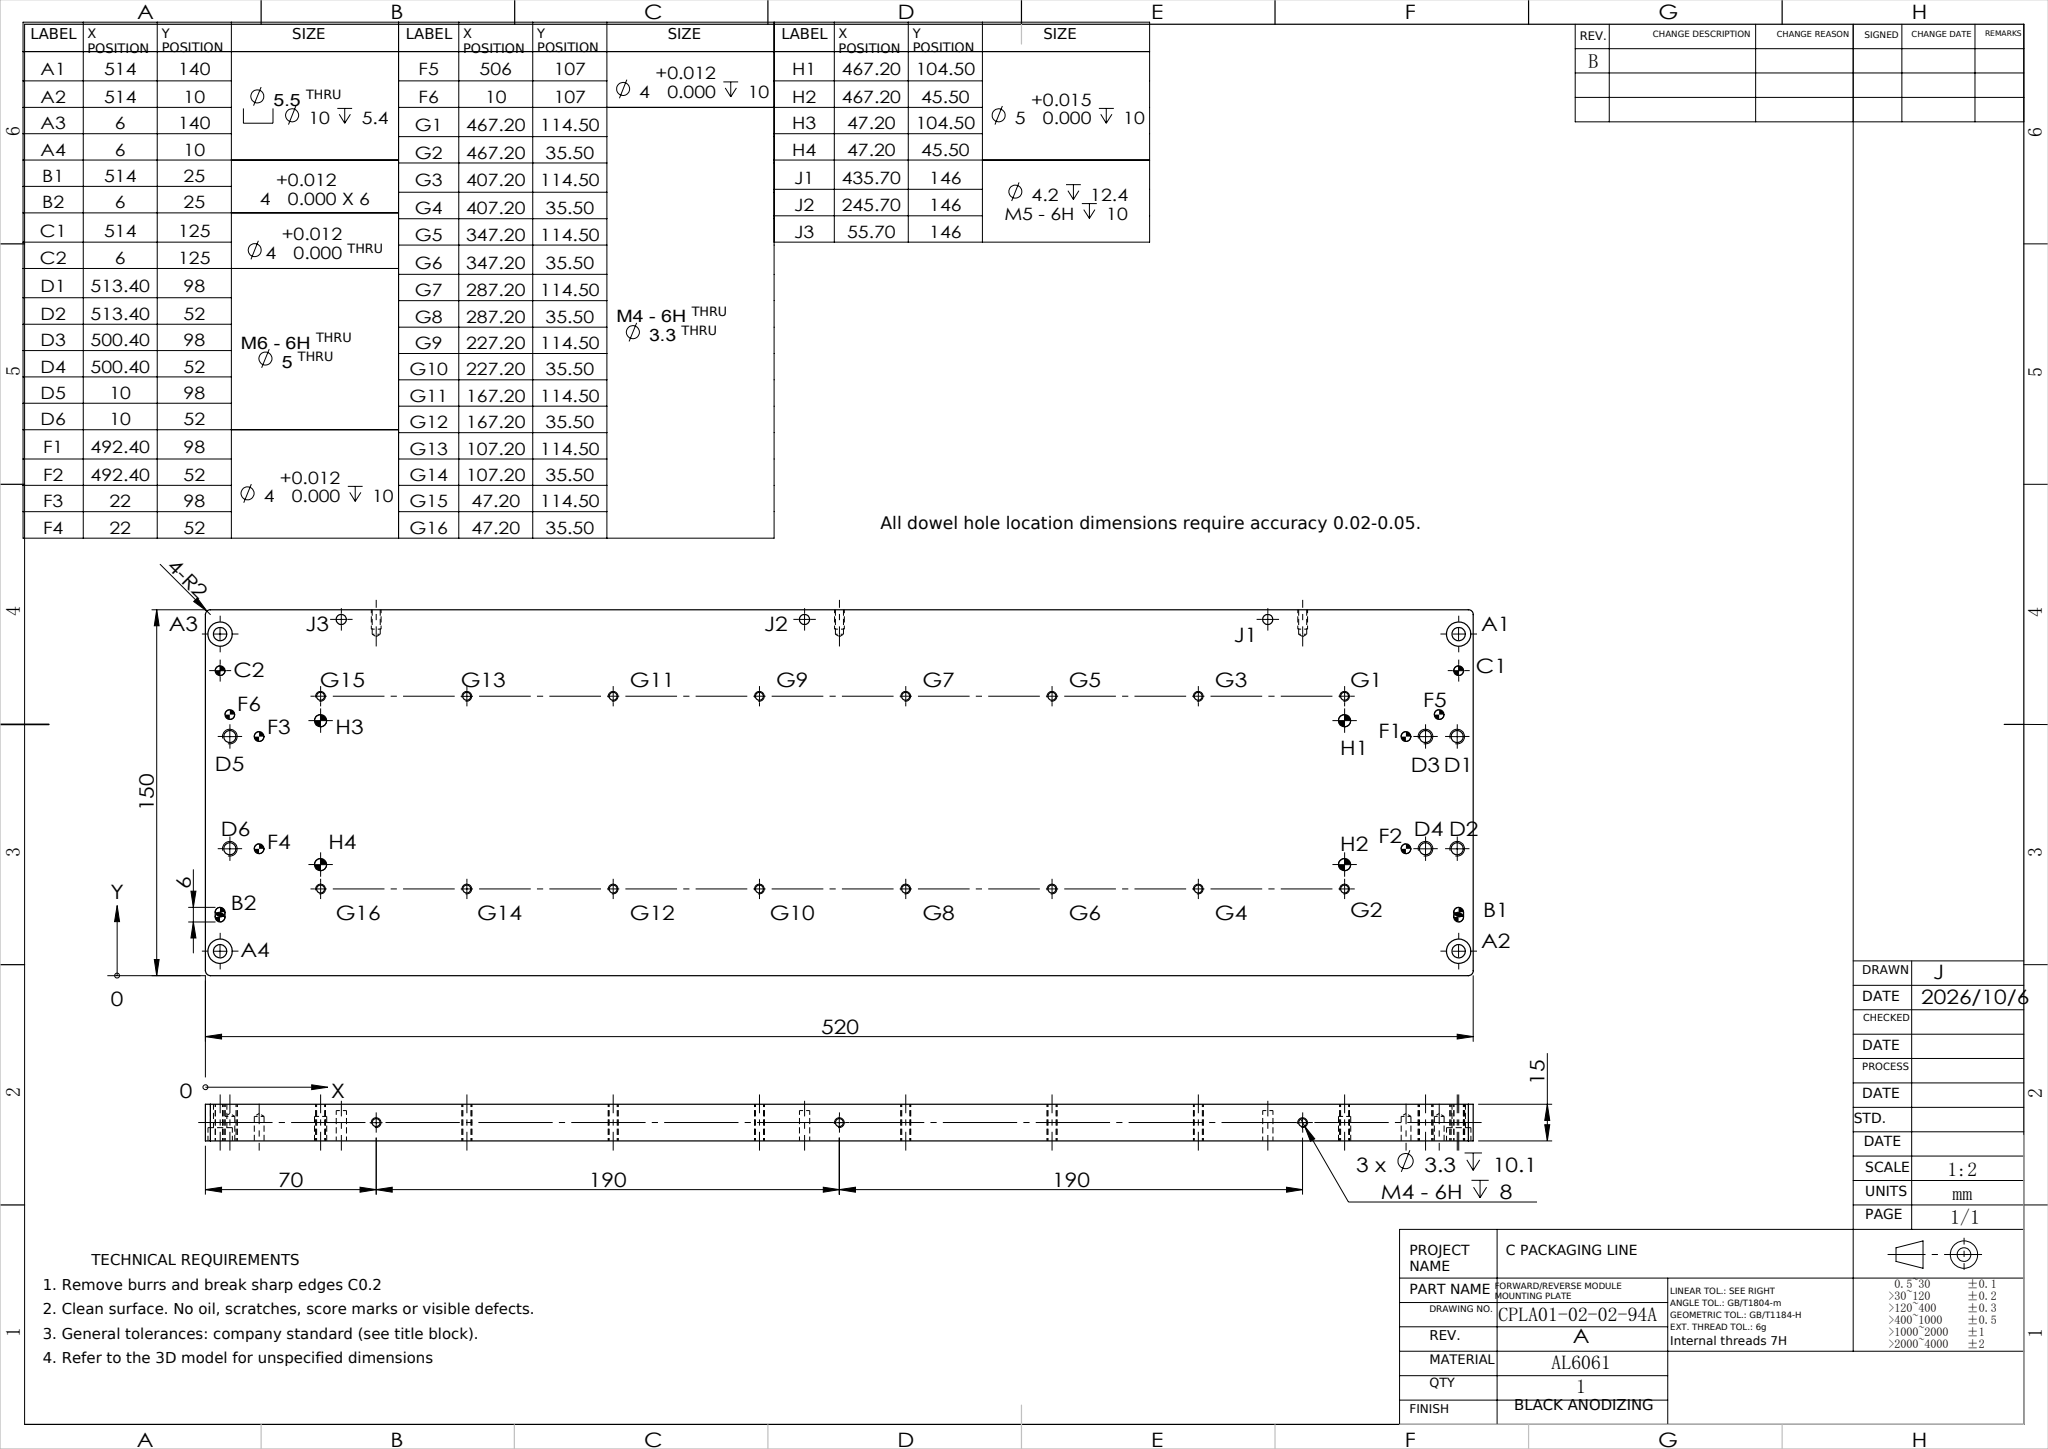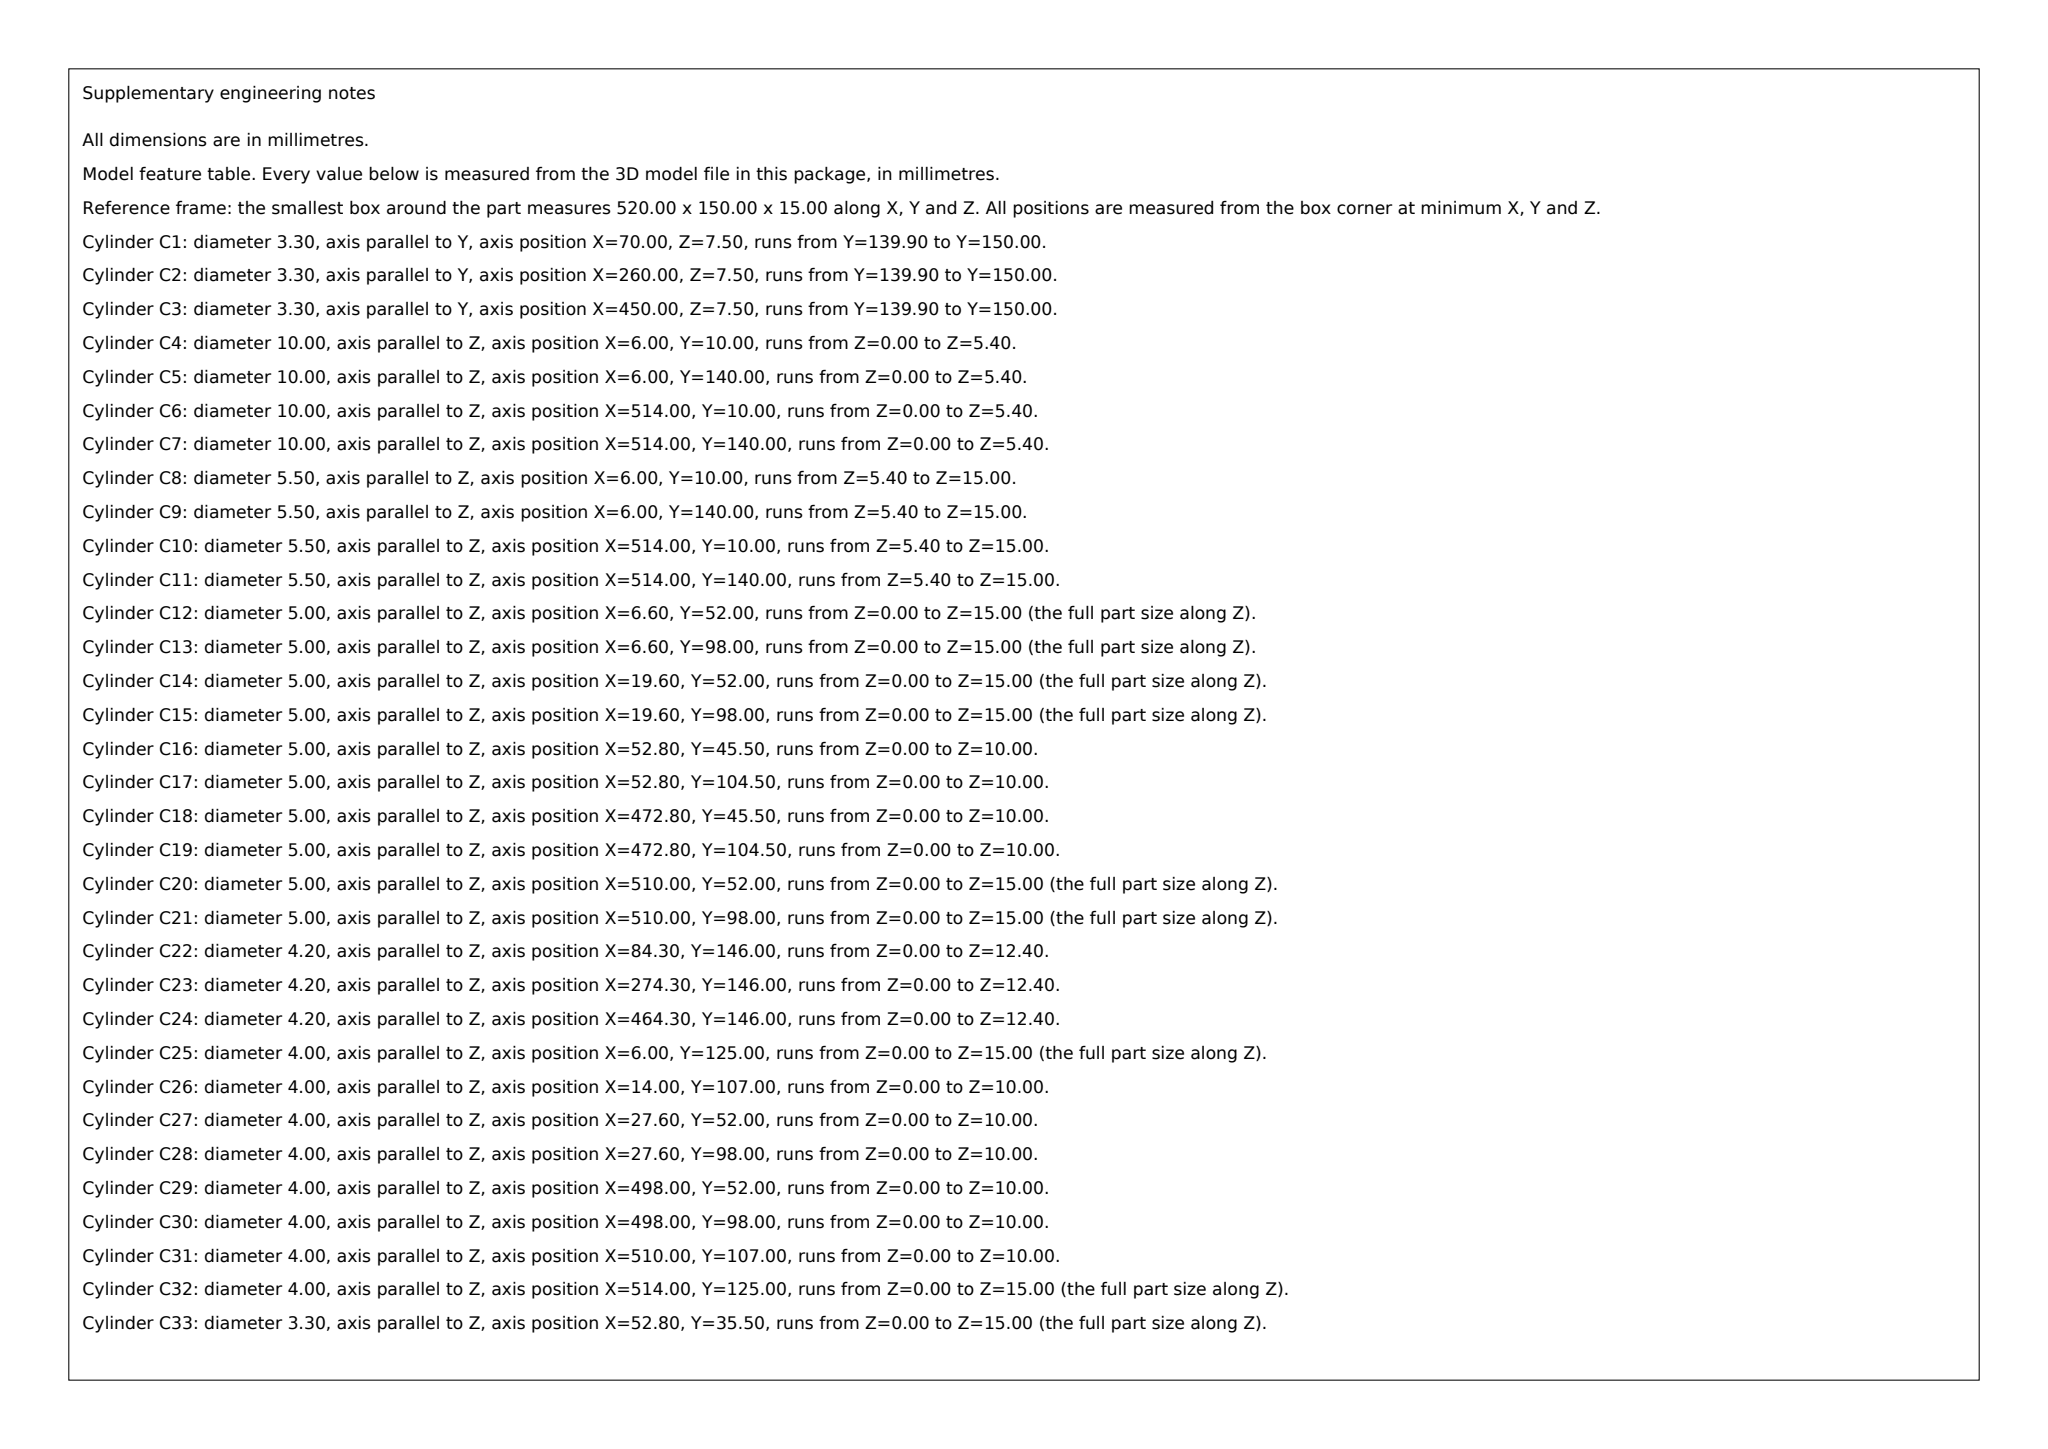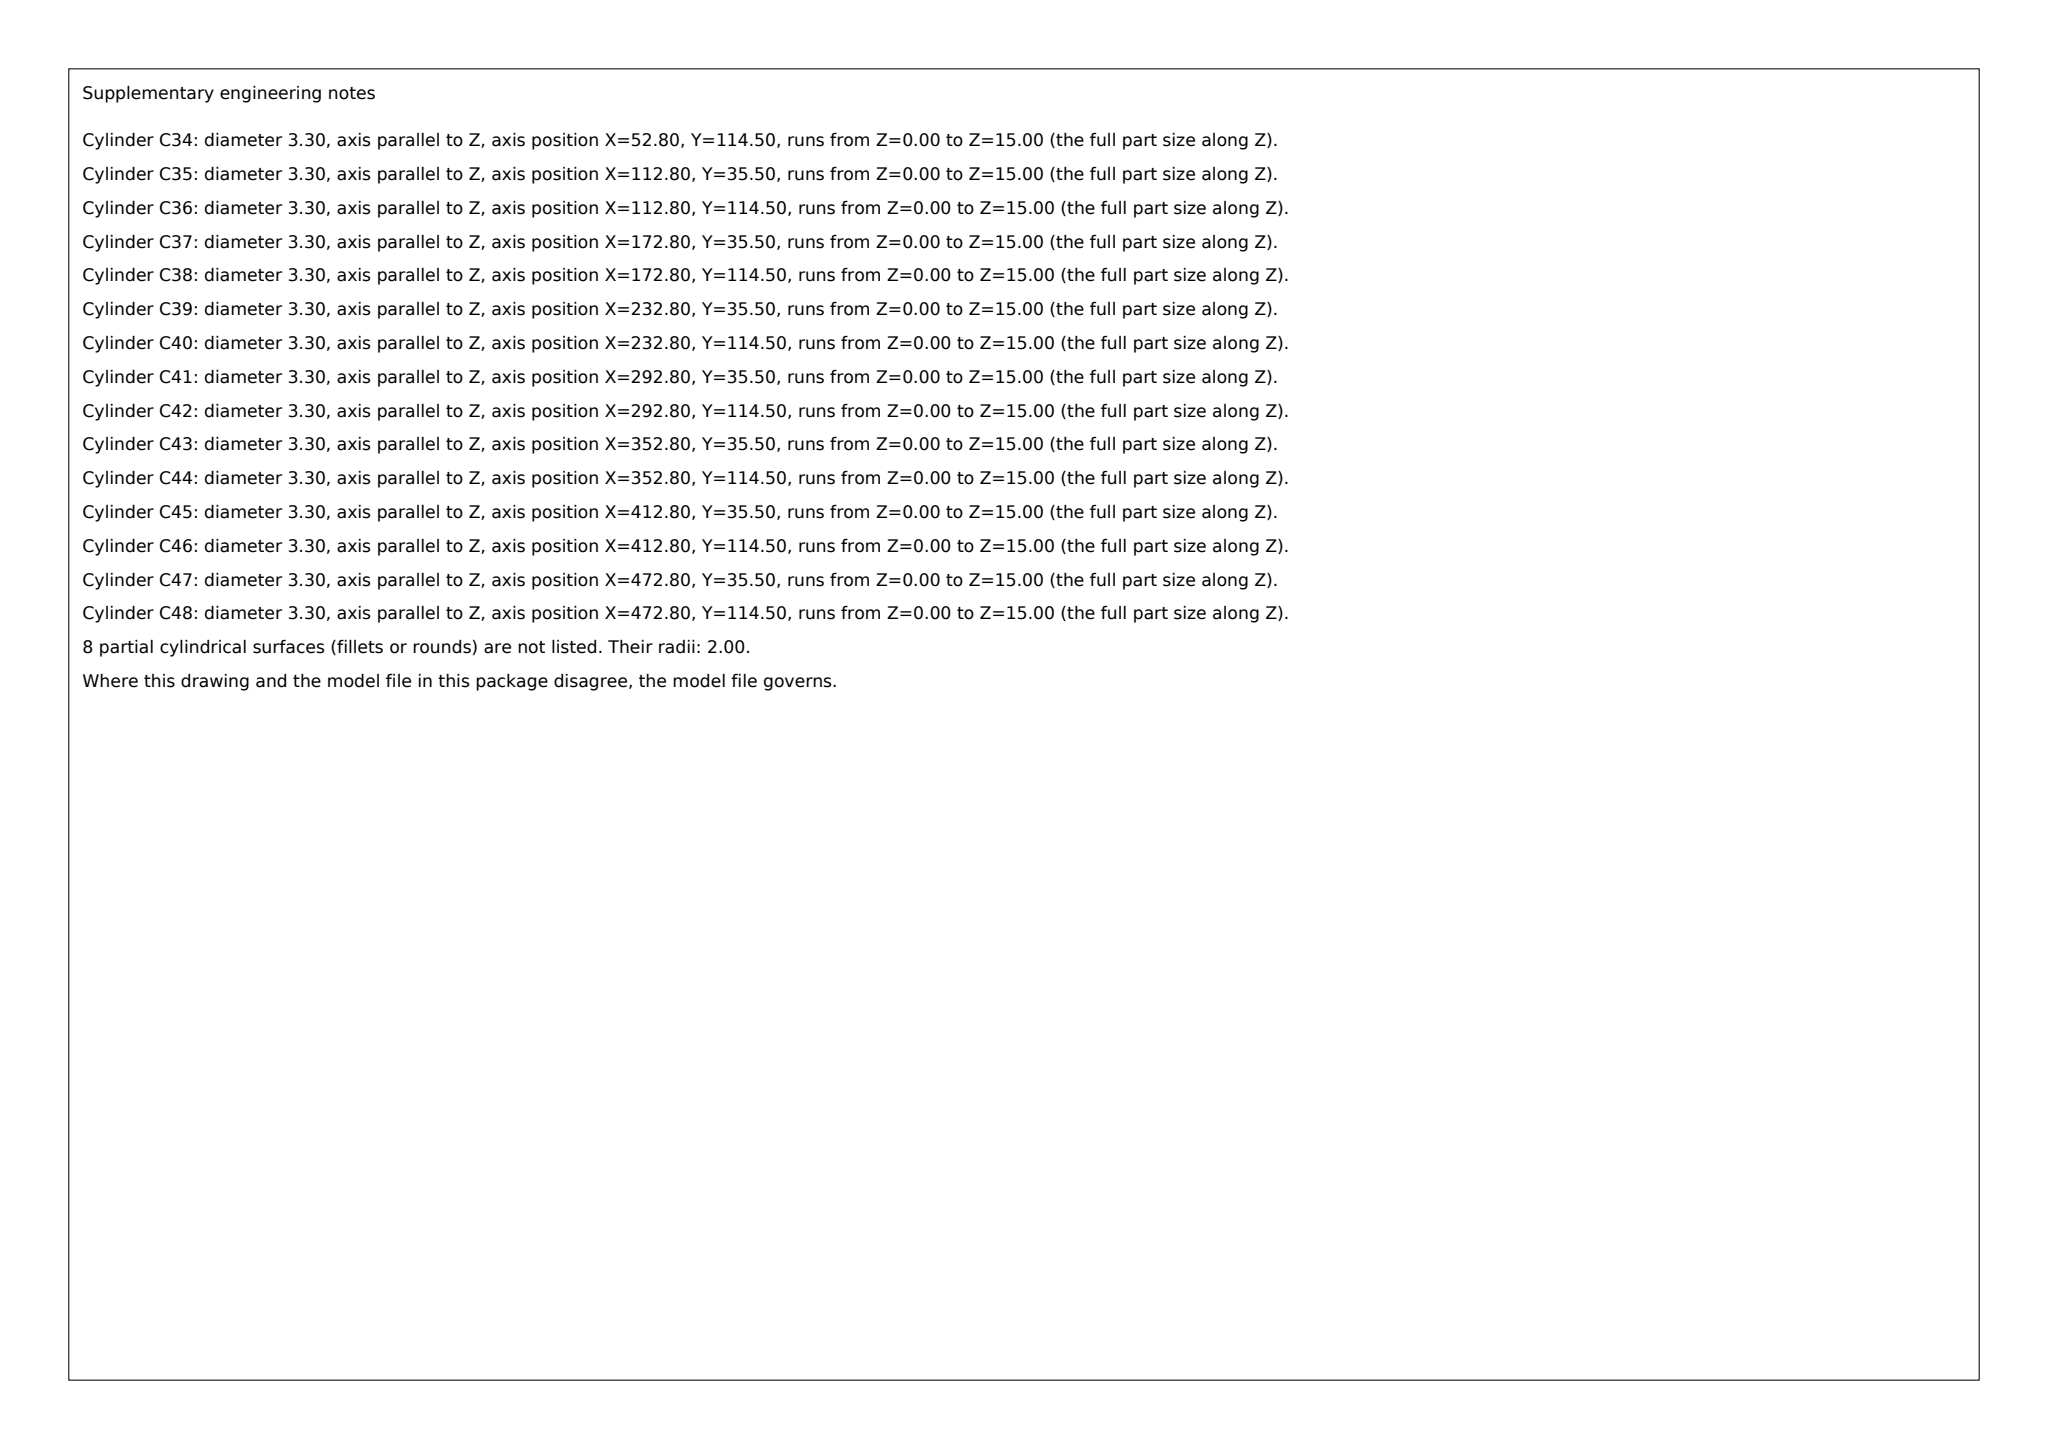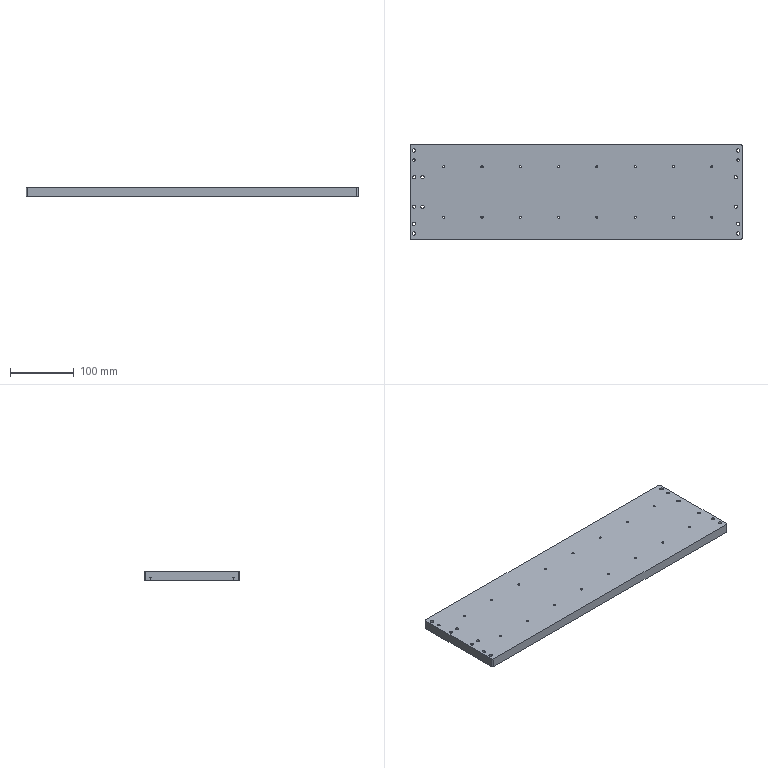Part | SolidWorks | mm | 1 solid | 143 faces | box 520 x 150 x 15 mm | volume 1160173 mm3 | cylinder 104 | plane 21 | cone 18 | commonest cylinder face diameters 3.3 x38 4 x24 5 x20 10 x8 5.5 x8 4.2 x6
build123d program:
from build123d import *

# Parameters (mm, degrees)
SKETCH1_W                                       = 520
SKETCH1_H                                       = 150
BOSS_EXTRUDE1_DEPTH                             = 7.5
FILLET1_R                                       = 2
M6_TAPPED_HOLE2_D                               = 5
M4_TAPPED_HOLE1_D                               = 3.3
LPATTERN1_COUNT                                 = 8
LPATTERN1_PITCH                                 = 60
M5_HEX_SOCKET_HEAD_CAP_SCREW_CBORE1_D           = 5.5
M5_HEX_SOCKET_HEAD_CAP_SCREW_CBORE1_CBORE_D     = 10
M5_HEX_SOCKET_HEAD_CAP_SCREW_CBORE1_CBORE_DEPTH = 5.4
M5_TAPPED_HOLE2_D                               = 4.2
M5_TAPPED_HOLE2_DEPTH                           = 12.4
F_5_0_MM_DOWEL_HOLE_1_D                         = 5
F_5_0_MM_DOWEL_HOLE_1_DEPTH                     = 10
F_5_0_MM_DOWEL_HOLE_2_D                         = 5
F_5_0_MM_DOWEL_HOLE_2_DEPTH                     = 10
F_4_0MM_DOWEL_HOLE_1_D                          = 4
F_4_0MM_DOWEL_HOLE_1_DEPTH                      = 10
F_4_0MM_DOWEL_HOLE_1_TIP                        = 1.202
M4_TAPPED_HOLE2_D                               = 3.3
M4_TAPPED_HOLE2_DEPTH                           = 10.1
M4_TAPPED_HOLE2_TIP                             = 0.9914
SKETCH48_R                                      = 2
CUT_EXTRUDE1_DEPTH                              = 272.017
F_4_0MM_DOWEL_HOLE_2_D                          = 4
F_4_0MM_DOWEL_HOLE_2_DEPTH                      = 10
F_4_0MM_DOWEL_HOLE_2_TIP                        = 1.202


with BuildPart() as part:
    # Sketch1 → Boss-Extrude1 (new, symmetric)
    with BuildSketch(Plane.XY):
        Rectangle(SKETCH1_W, SKETCH1_H)
    extrude(amount=BOSS_EXTRUDE1_DEPTH, both=True)

    # Fillet1
    fillet1_edges = [part.edges().sort_by_distance(p)[0] for p in [
        (260, -75, 0),
        (-260, -75, 0),
        (-260, 75, 0),
        (260, 75, 0),
    ]]
    fillet(fillet1_edges, radius=FILLET1_R)

    # M6 Tapped Hole2 (through all)
    with Locations(Plane(origin=(0, 0, -7.5), x_dir=(-1, 0, 0), z_dir=(0, 0, -1))):
        with Locations((-250, 23), (-250, -23), (240.4, 23), (253.4, 23), (253.4, -23), (240.4, -23)):
            Hole(M6_TAPPED_HOLE2_D / 2)

    # M4 Tapped Hole1 (through all)
    with Locations(Plane(origin=(0, 0, -7.5), x_dir=(-1, 0, 0), z_dir=(0, 0, -1))):
        with Locations((-212.8, 39.5), (-212.8, -39.5)):
            m4_tapped_hole1 = Hole(M4_TAPPED_HOLE1_D / 2)

    # LPattern1: M4 Tapped Hole1 ×8
    with Locations(*[(-i * LPATTERN1_PITCH, 0, 0) for i in range(1, LPATTERN1_COUNT)]):
        add(m4_tapped_hole1, mode=Mode.SUBTRACT)

    # M5 Hex Socket Head Cap Screw CBORE1 (through all)
    with Locations(Plane(origin=(0, 0, -7.5), x_dir=(-1, 0, 0), z_dir=(0, 0, -1))):
        with Locations((-254, 65), (254, 65), (-254, -65), (254, -65)):
            CounterBoreHole(M5_HEX_SOCKET_HEAD_CAP_SCREW_CBORE1_D / 2, M5_HEX_SOCKET_HEAD_CAP_SCREW_CBORE1_CBORE_D / 2, M5_HEX_SOCKET_HEAD_CAP_SCREW_CBORE1_CBORE_DEPTH)

    # M5 Tapped Hole2
    with Locations(Plane(origin=(0, 0, -7.5), x_dir=(-1, 0, 0), z_dir=(0, 0, -1))):
        with Locations((175.704, 71), (-14.296, 71), (-204.296, 71)):
            Hole(M5_TAPPED_HOLE2_D / 2, depth=M5_TAPPED_HOLE2_DEPTH)

    # 5.0 mm Dowel Hole 1
    with Locations(Plane(origin=(0, 0, -7.5), x_dir=(-1, 0, 0), z_dir=(0, 0, -1))):
        with Locations((207.2, -29.5), (-212.8, -29.5)):
            Hole(F_5_0_MM_DOWEL_HOLE_1_D / 2, depth=F_5_0_MM_DOWEL_HOLE_1_DEPTH)

    # 5.0 mm Dowel Hole 2
    with Locations(Plane(origin=(0, 0, -7.5), x_dir=(-1, 0, 0), z_dir=(0, 0, -1))):
        with Locations((207.2, 29.5), (-212.8, 29.5)):
            Hole(F_5_0_MM_DOWEL_HOLE_2_D / 2, depth=F_5_0_MM_DOWEL_HOLE_2_DEPTH)

    # 4.0mm Dowel Hole 1
    with Locations(Plane(origin=(0, 0, -7.5), x_dir=(-1, 0, 0), z_dir=(0, 0, -1))):
        with Locations((-238, 23), (-238, -23), (232.4, -23), (232.4, 23)):
            Hole(F_4_0MM_DOWEL_HOLE_1_D / 2, depth=F_4_0MM_DOWEL_HOLE_1_DEPTH)
            with Locations((0, 0, -(F_4_0MM_DOWEL_HOLE_1_DEPTH + F_4_0MM_DOWEL_HOLE_1_TIP / 2))):  # 118° drill point
                Cone(0, F_4_0MM_DOWEL_HOLE_1_D / 2, F_4_0MM_DOWEL_HOLE_1_TIP, mode=Mode.SUBTRACT)

    # M4 Tapped Hole2
    with Locations(Plane(origin=(0, 75, 0), x_dir=(1, 0, 0), z_dir=(0, 1, 0))):
        with Locations((190, 0), (0, 0), (-190, 0)):
            Hole(M4_TAPPED_HOLE2_D / 2, depth=M4_TAPPED_HOLE2_DEPTH)
            with Locations((0, 0, -(M4_TAPPED_HOLE2_DEPTH + M4_TAPPED_HOLE2_TIP / 2))):  # 118° drill point
                Cone(0, M4_TAPPED_HOLE2_D / 2, M4_TAPPED_HOLE2_TIP, mode=Mode.SUBTRACT)

    # Sketch48 → Cut-Extrude1 (cut, through all)
    with BuildSketch(Plane(origin=(0, 0, -7.5), x_dir=(-1, 0, 0), z_dir=(0, 0, -1))):
        with Locations((-254, 50)):
            Circle(SKETCH48_R)
        with BuildLine():
            Line((-252, -49), (-252, -51))
            ThreePointArc((-252, -51), (-254, -53), (-256, -51))
            Line((-256, -51), (-256, -49))
            ThreePointArc((-256, -49), (-254, -47), (-252, -49))
        make_face()
    cut_extrude1 = extrude(amount=-CUT_EXTRUDE1_DEPTH, mode=Mode.SUBTRACT)

    # Mirror1: Cut-Extrude1 across plane
    add(cut_extrude1.mirror(Plane(origin=(0, 0, 0), x_dir=(0, 0, 1), z_dir=(1, 0, 0))), mode=Mode.SUBTRACT)

    # 4.0mm Dowel Hole 2
    with Locations(Plane(origin=(0, 0, -7.5), x_dir=(-1, 0, 0), z_dir=(0, 0, -1))):
        with Locations((246, 32), (-250, 32)):
            Hole(F_4_0MM_DOWEL_HOLE_2_D / 2, depth=F_4_0MM_DOWEL_HOLE_2_DEPTH)
            with Locations((0, 0, -(F_4_0MM_DOWEL_HOLE_2_DEPTH + F_4_0MM_DOWEL_HOLE_2_TIP / 2))):  # 118° drill point
                Cone(0, F_4_0MM_DOWEL_HOLE_2_D / 2, F_4_0MM_DOWEL_HOLE_2_TIP, mode=Mode.SUBTRACT)


solid = part.part